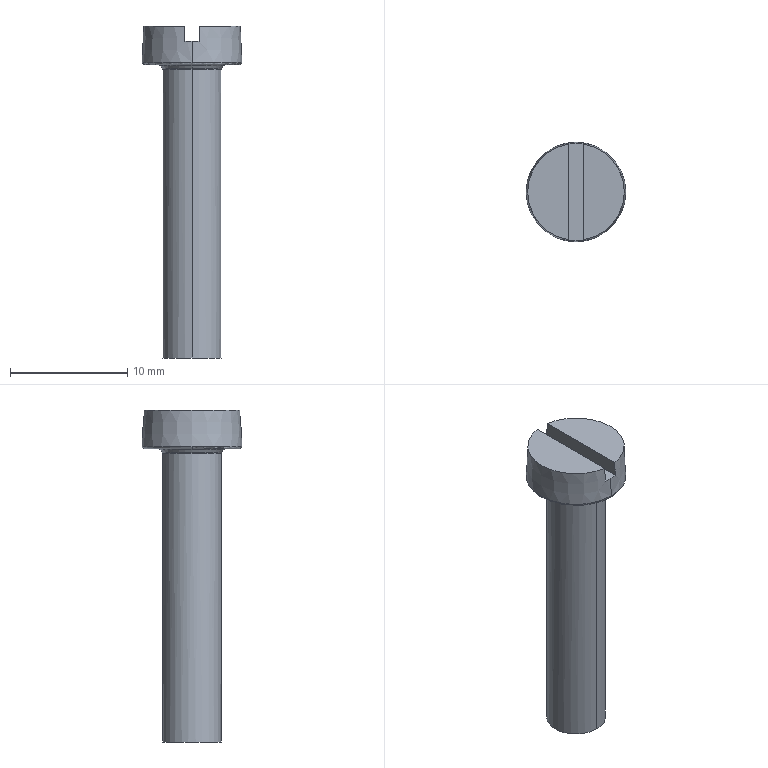Component | NX | SCREW_M5X25_2 | 1 solid | 19 faces | volume 660 mm3 | plane 7 | torus 6 | cone 4 | cylinder 2 | commonest cylinder face diameters 5 x2